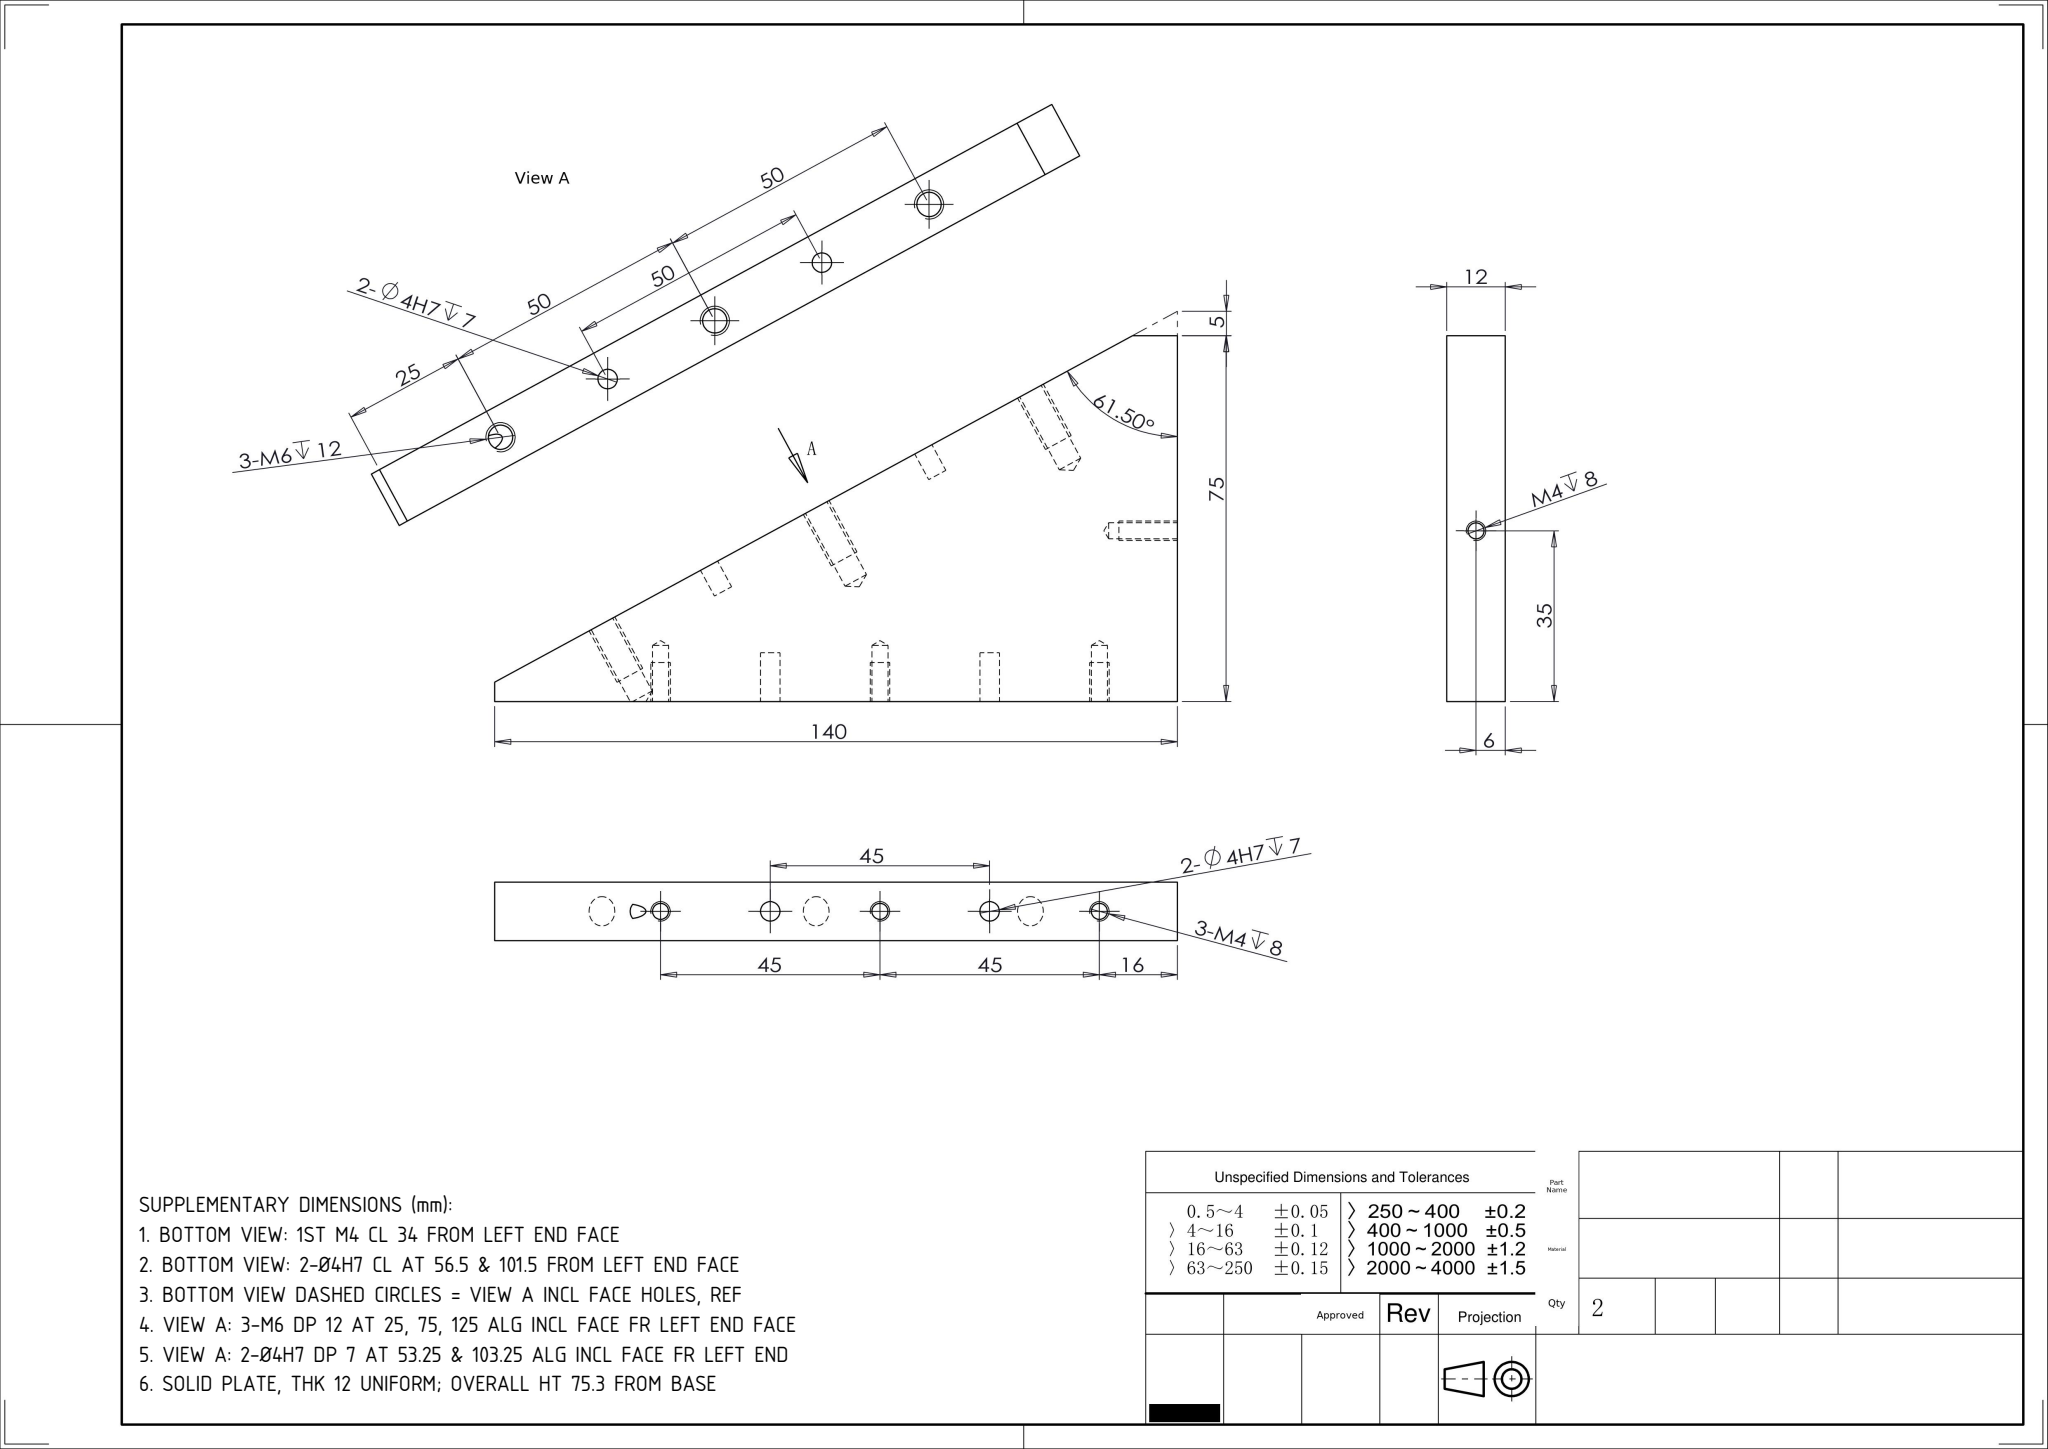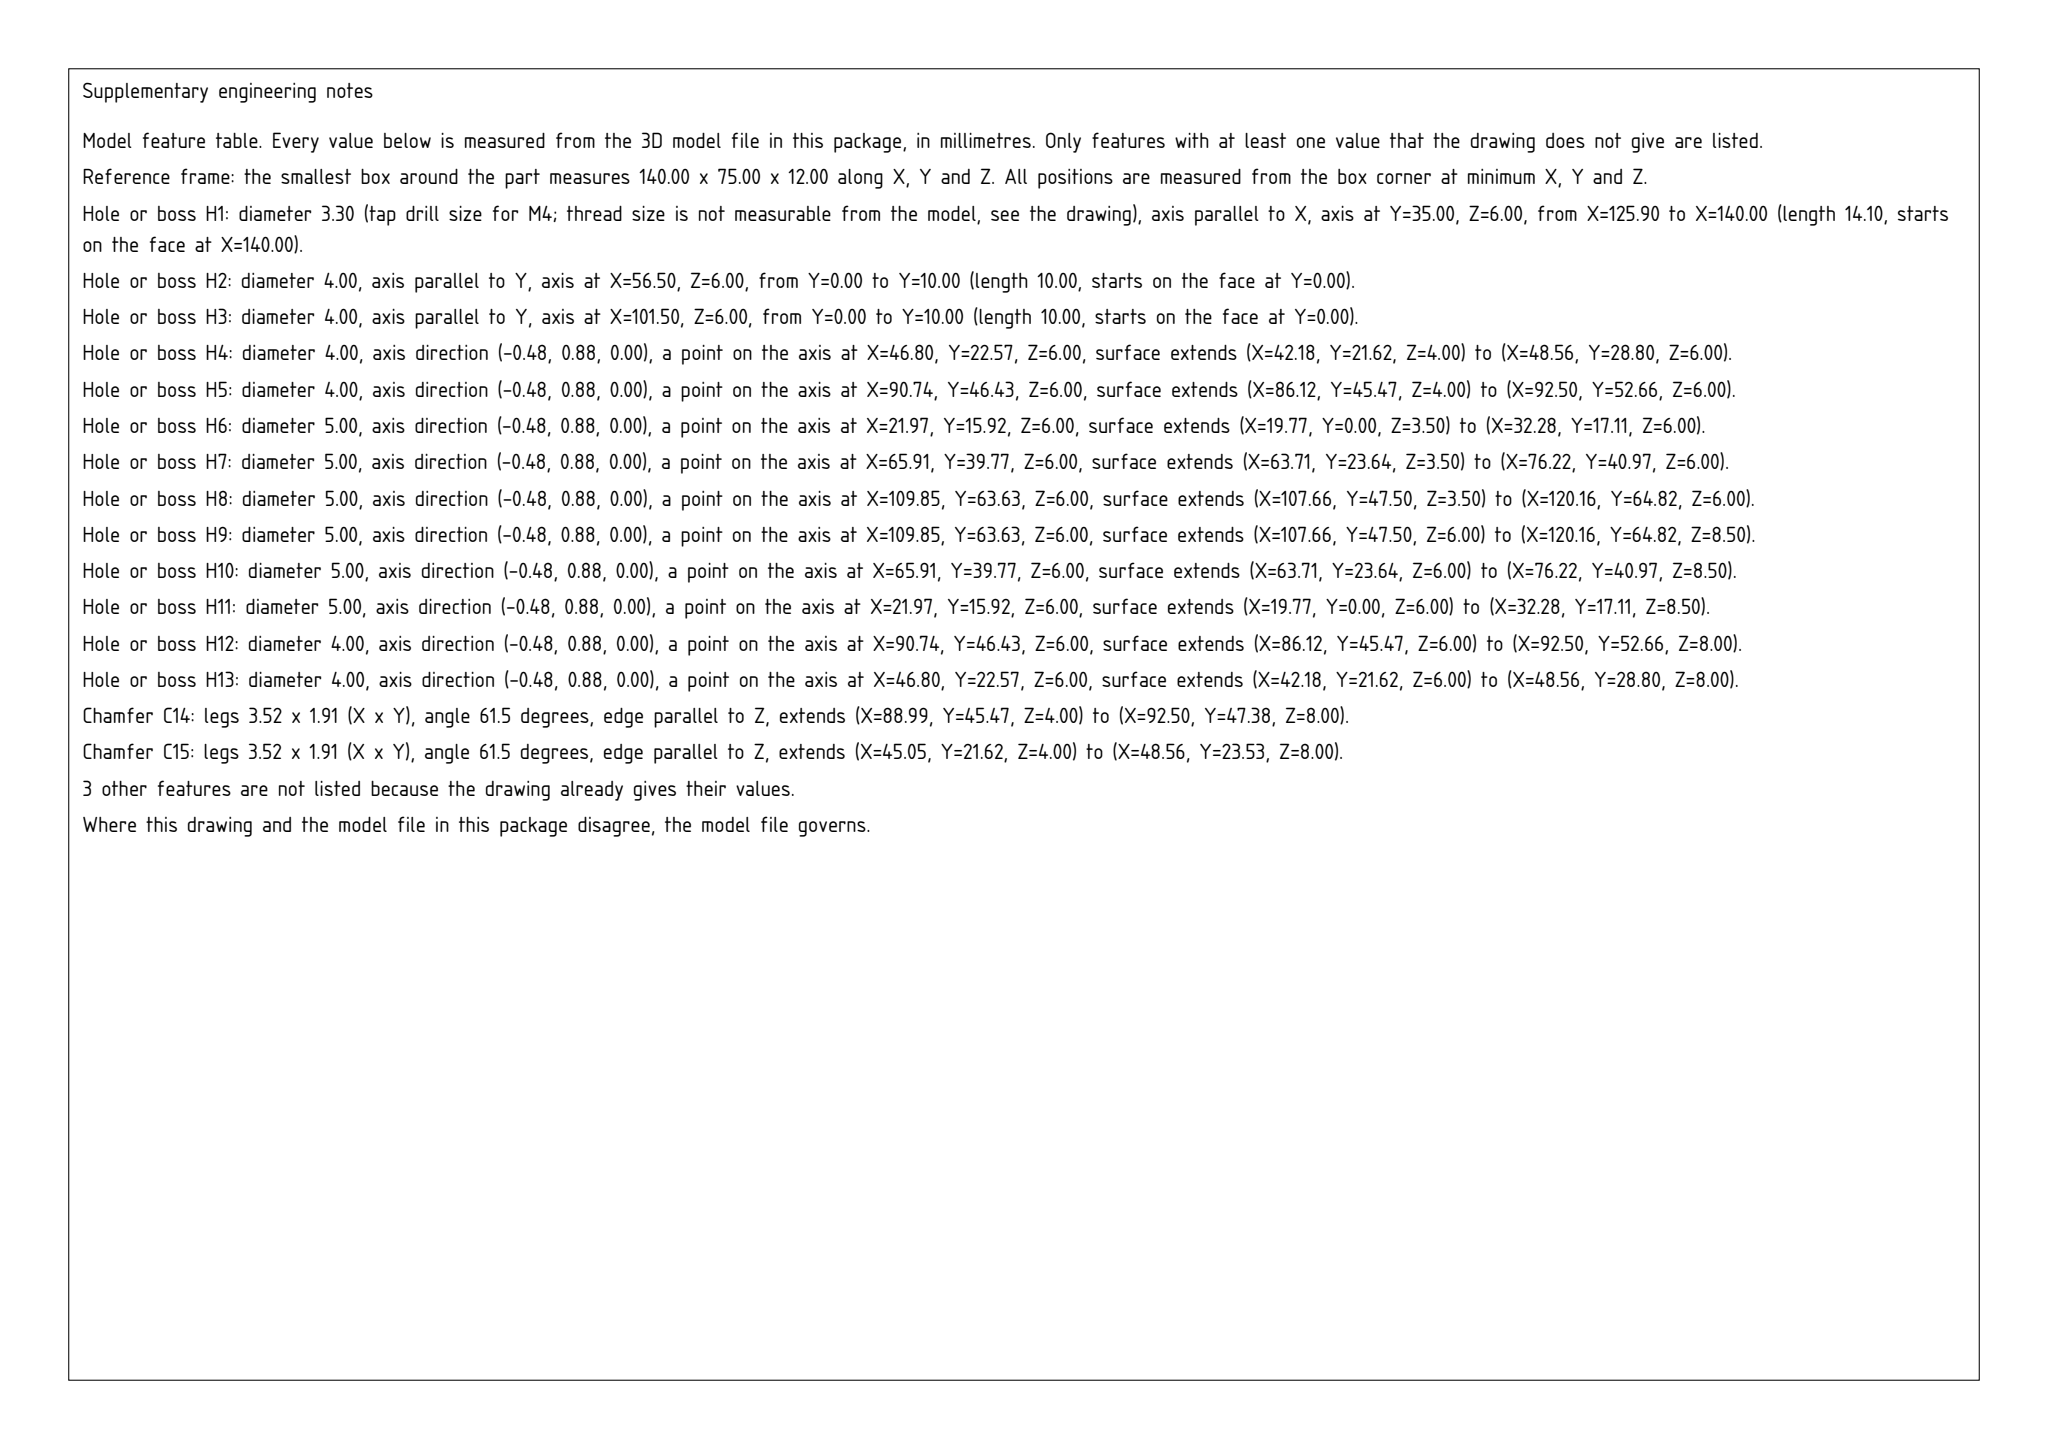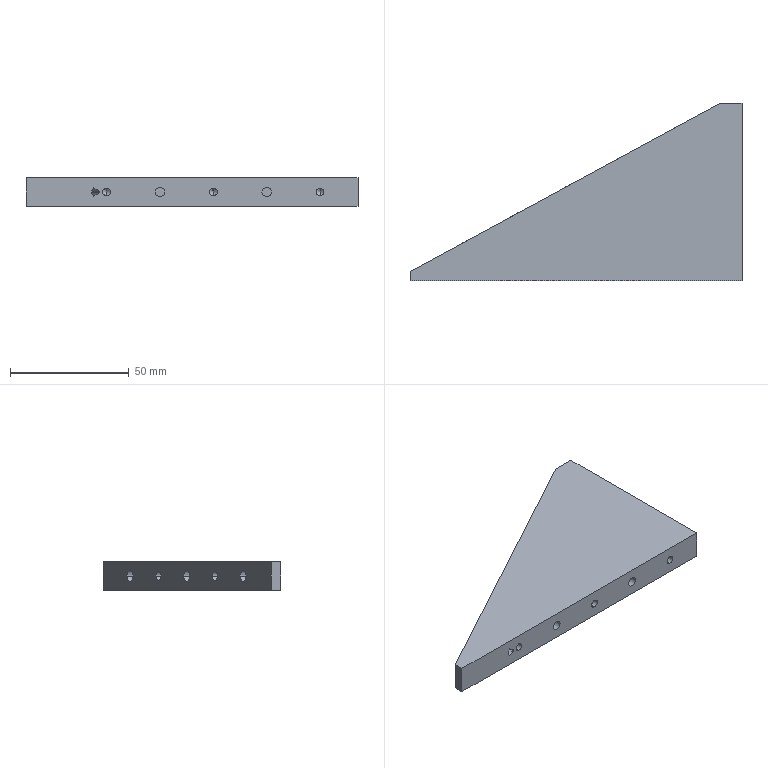Part | SolidWorks | mm | 1 solid | 46 faces | box 140 x 75 x 12 mm | volume 68413 mm3 | cylinder 22 | cone 13 | plane 11 | commonest cylinder face diameters 4 x8 3.3 x8 5 x6